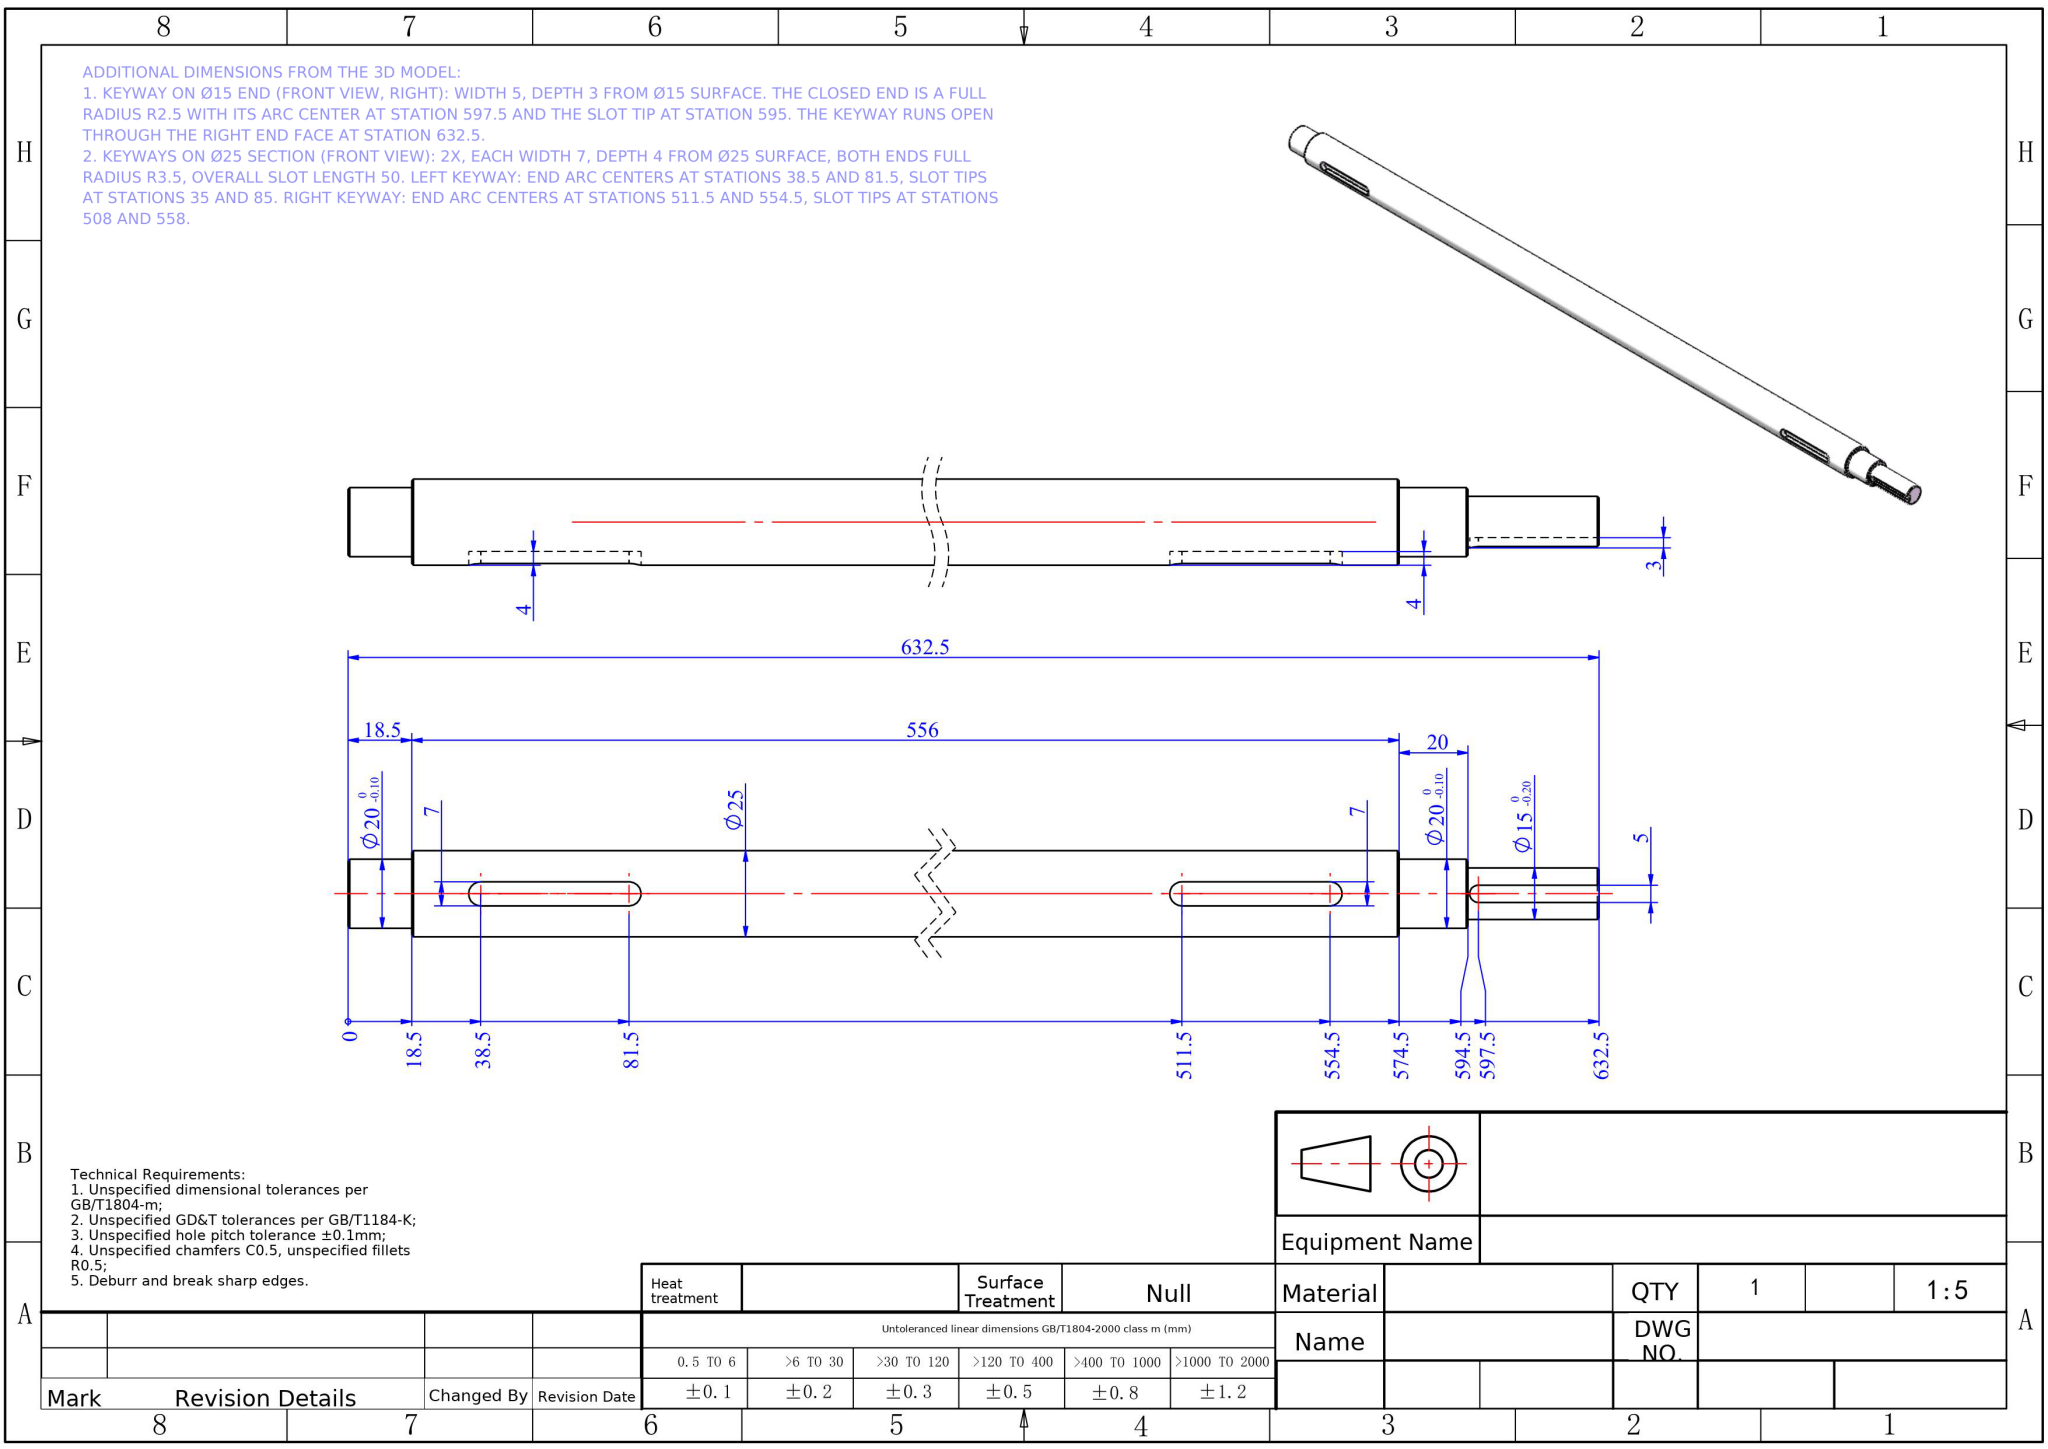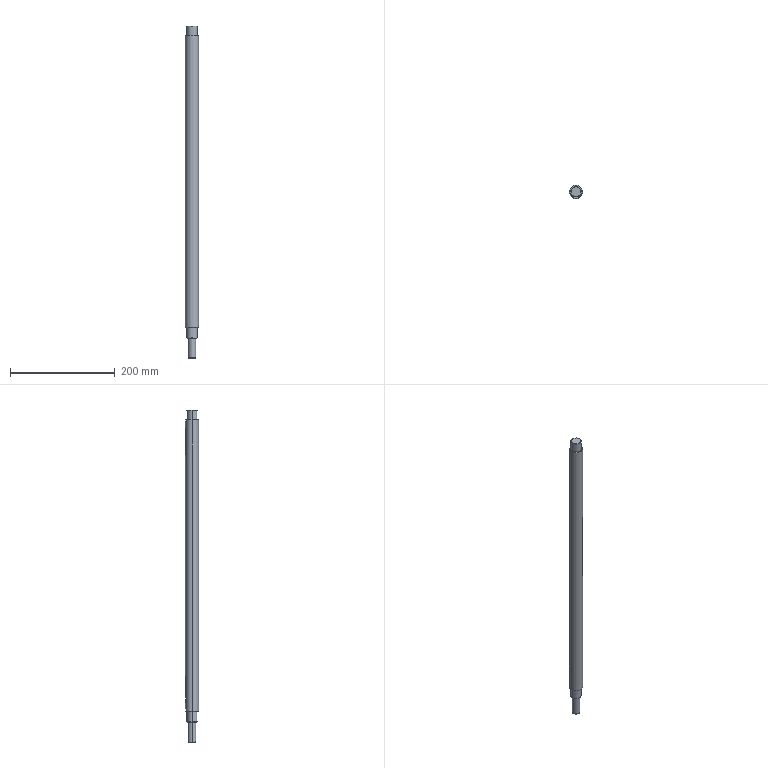Part | NX | mm | 1 solid | 41 faces | box 25 x 25 x 632.5 mm | volume 288561 mm3 | cylinder 16 | plane 14 | cone 11 | commonest cylinder face diameters 7 x6 20 x4 5 x2 15 x2 25 x2